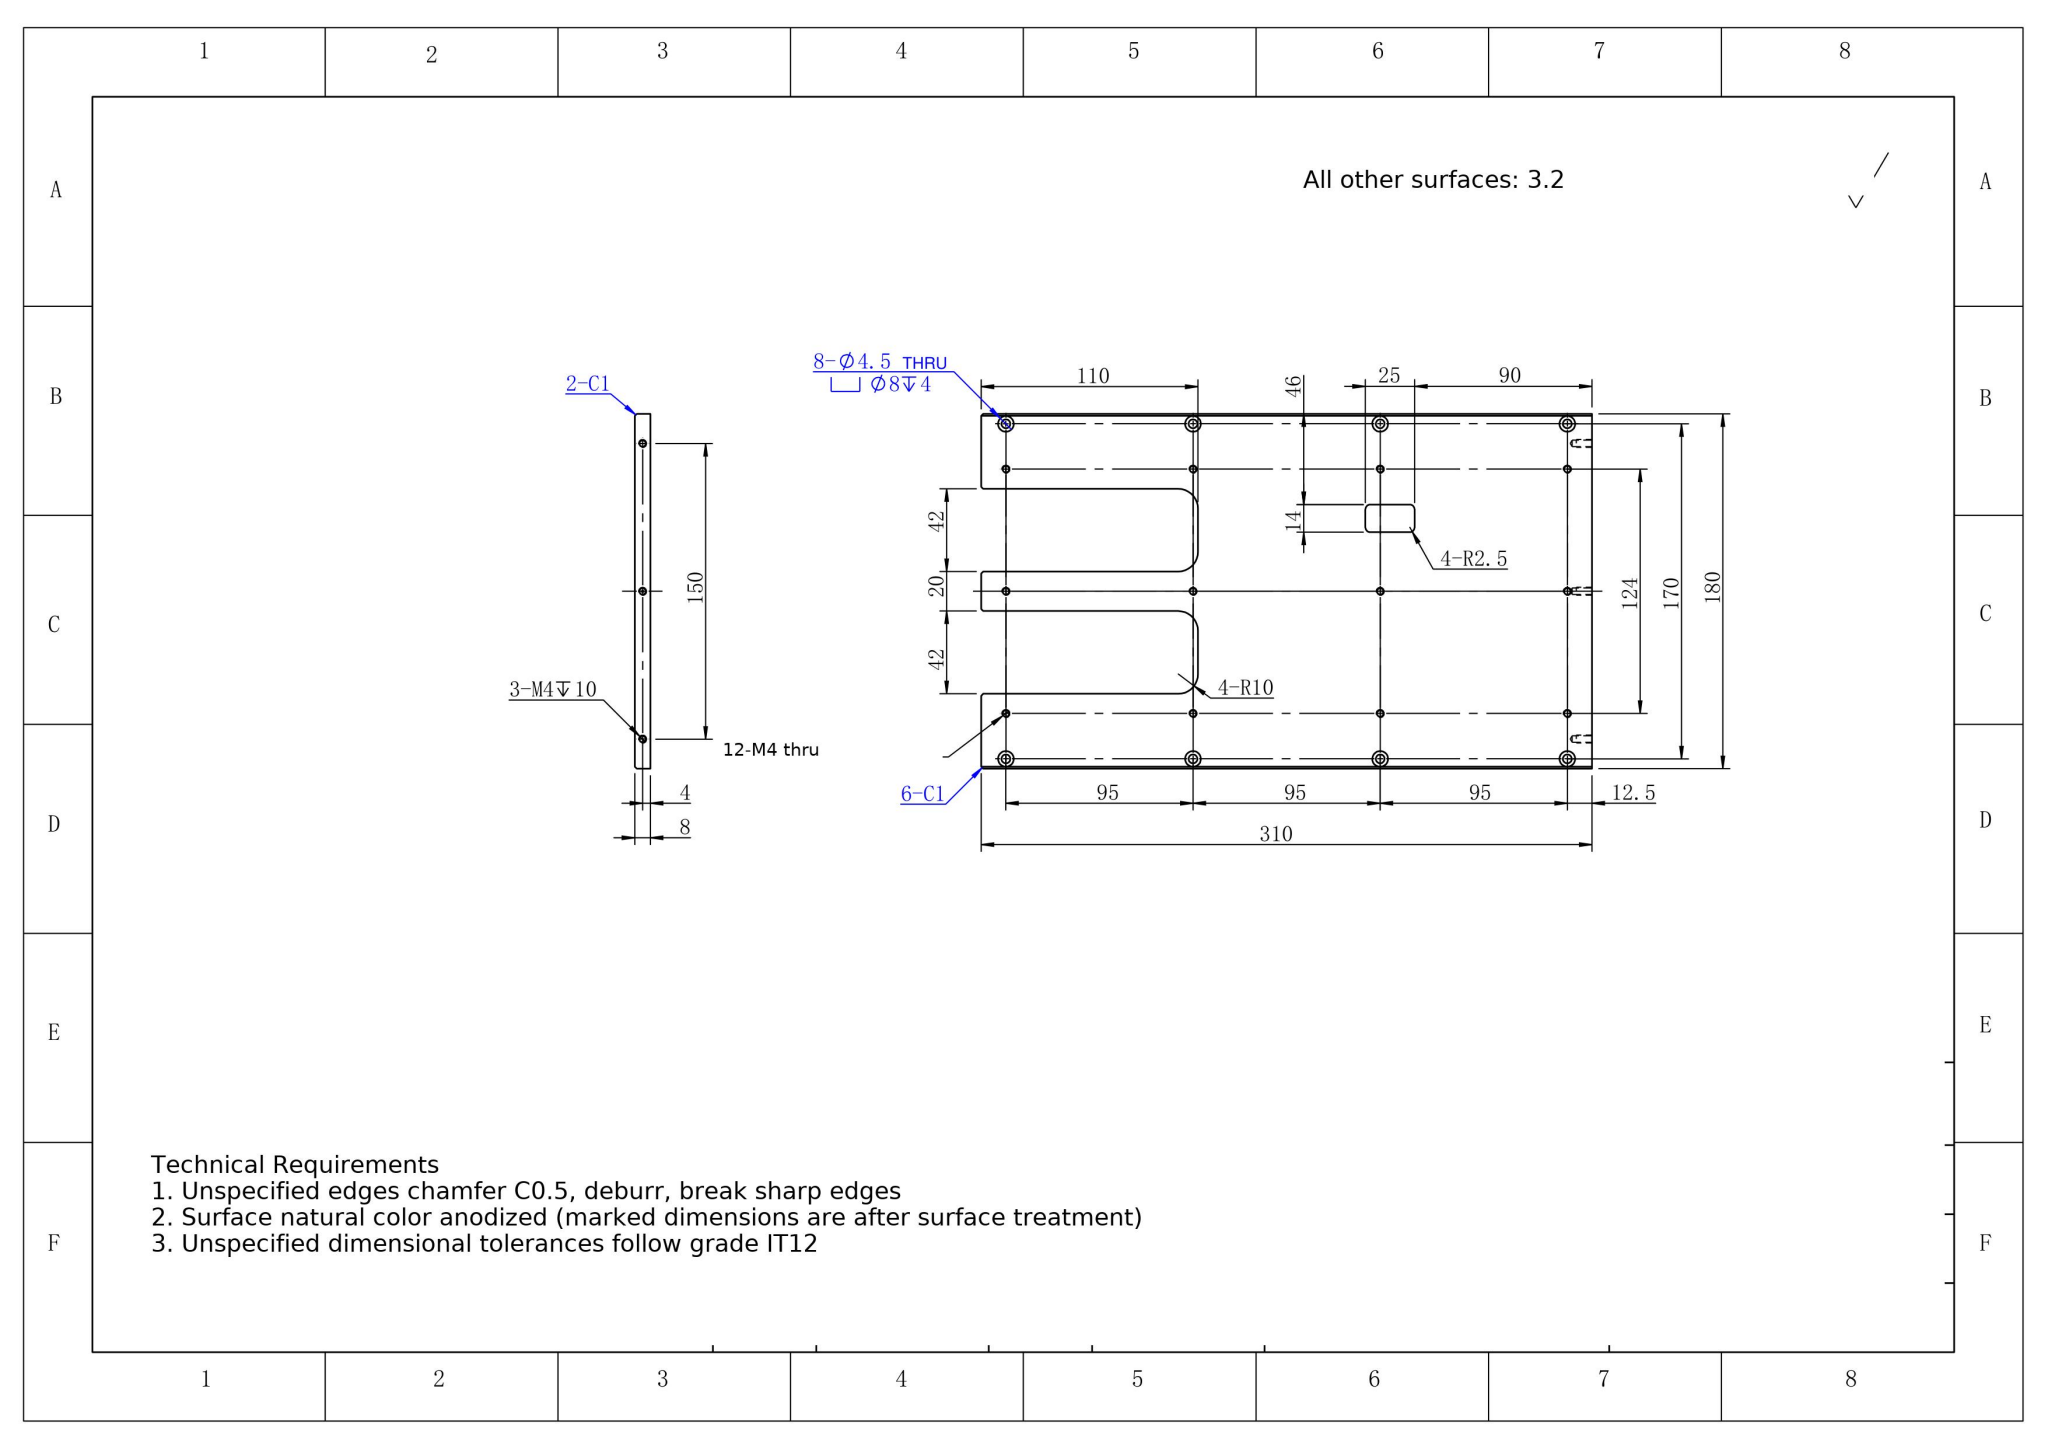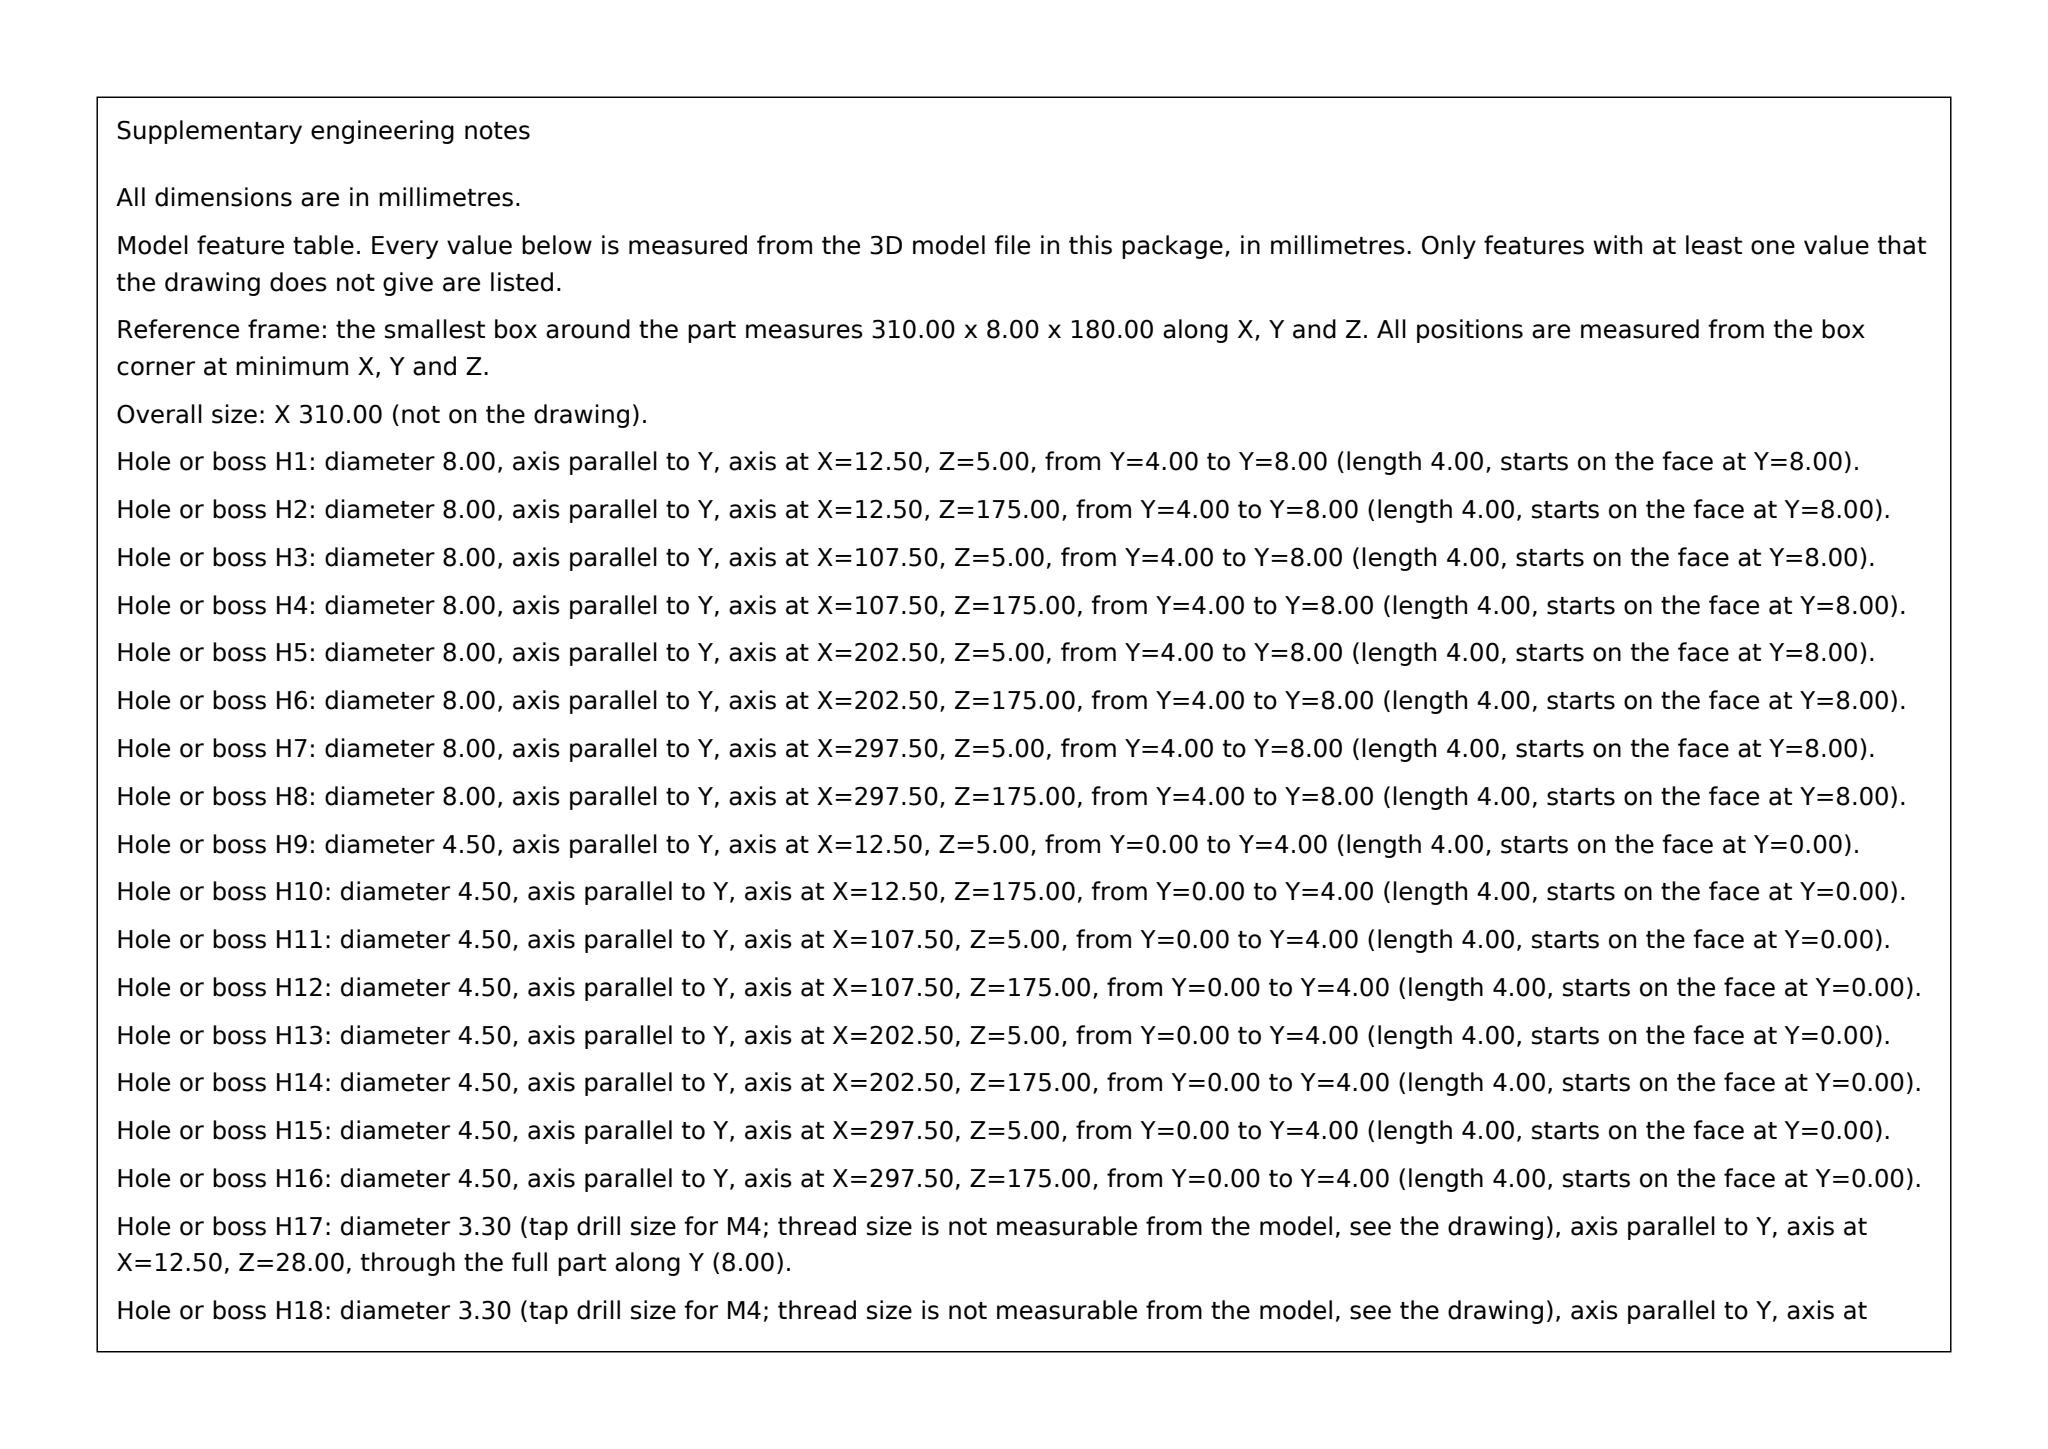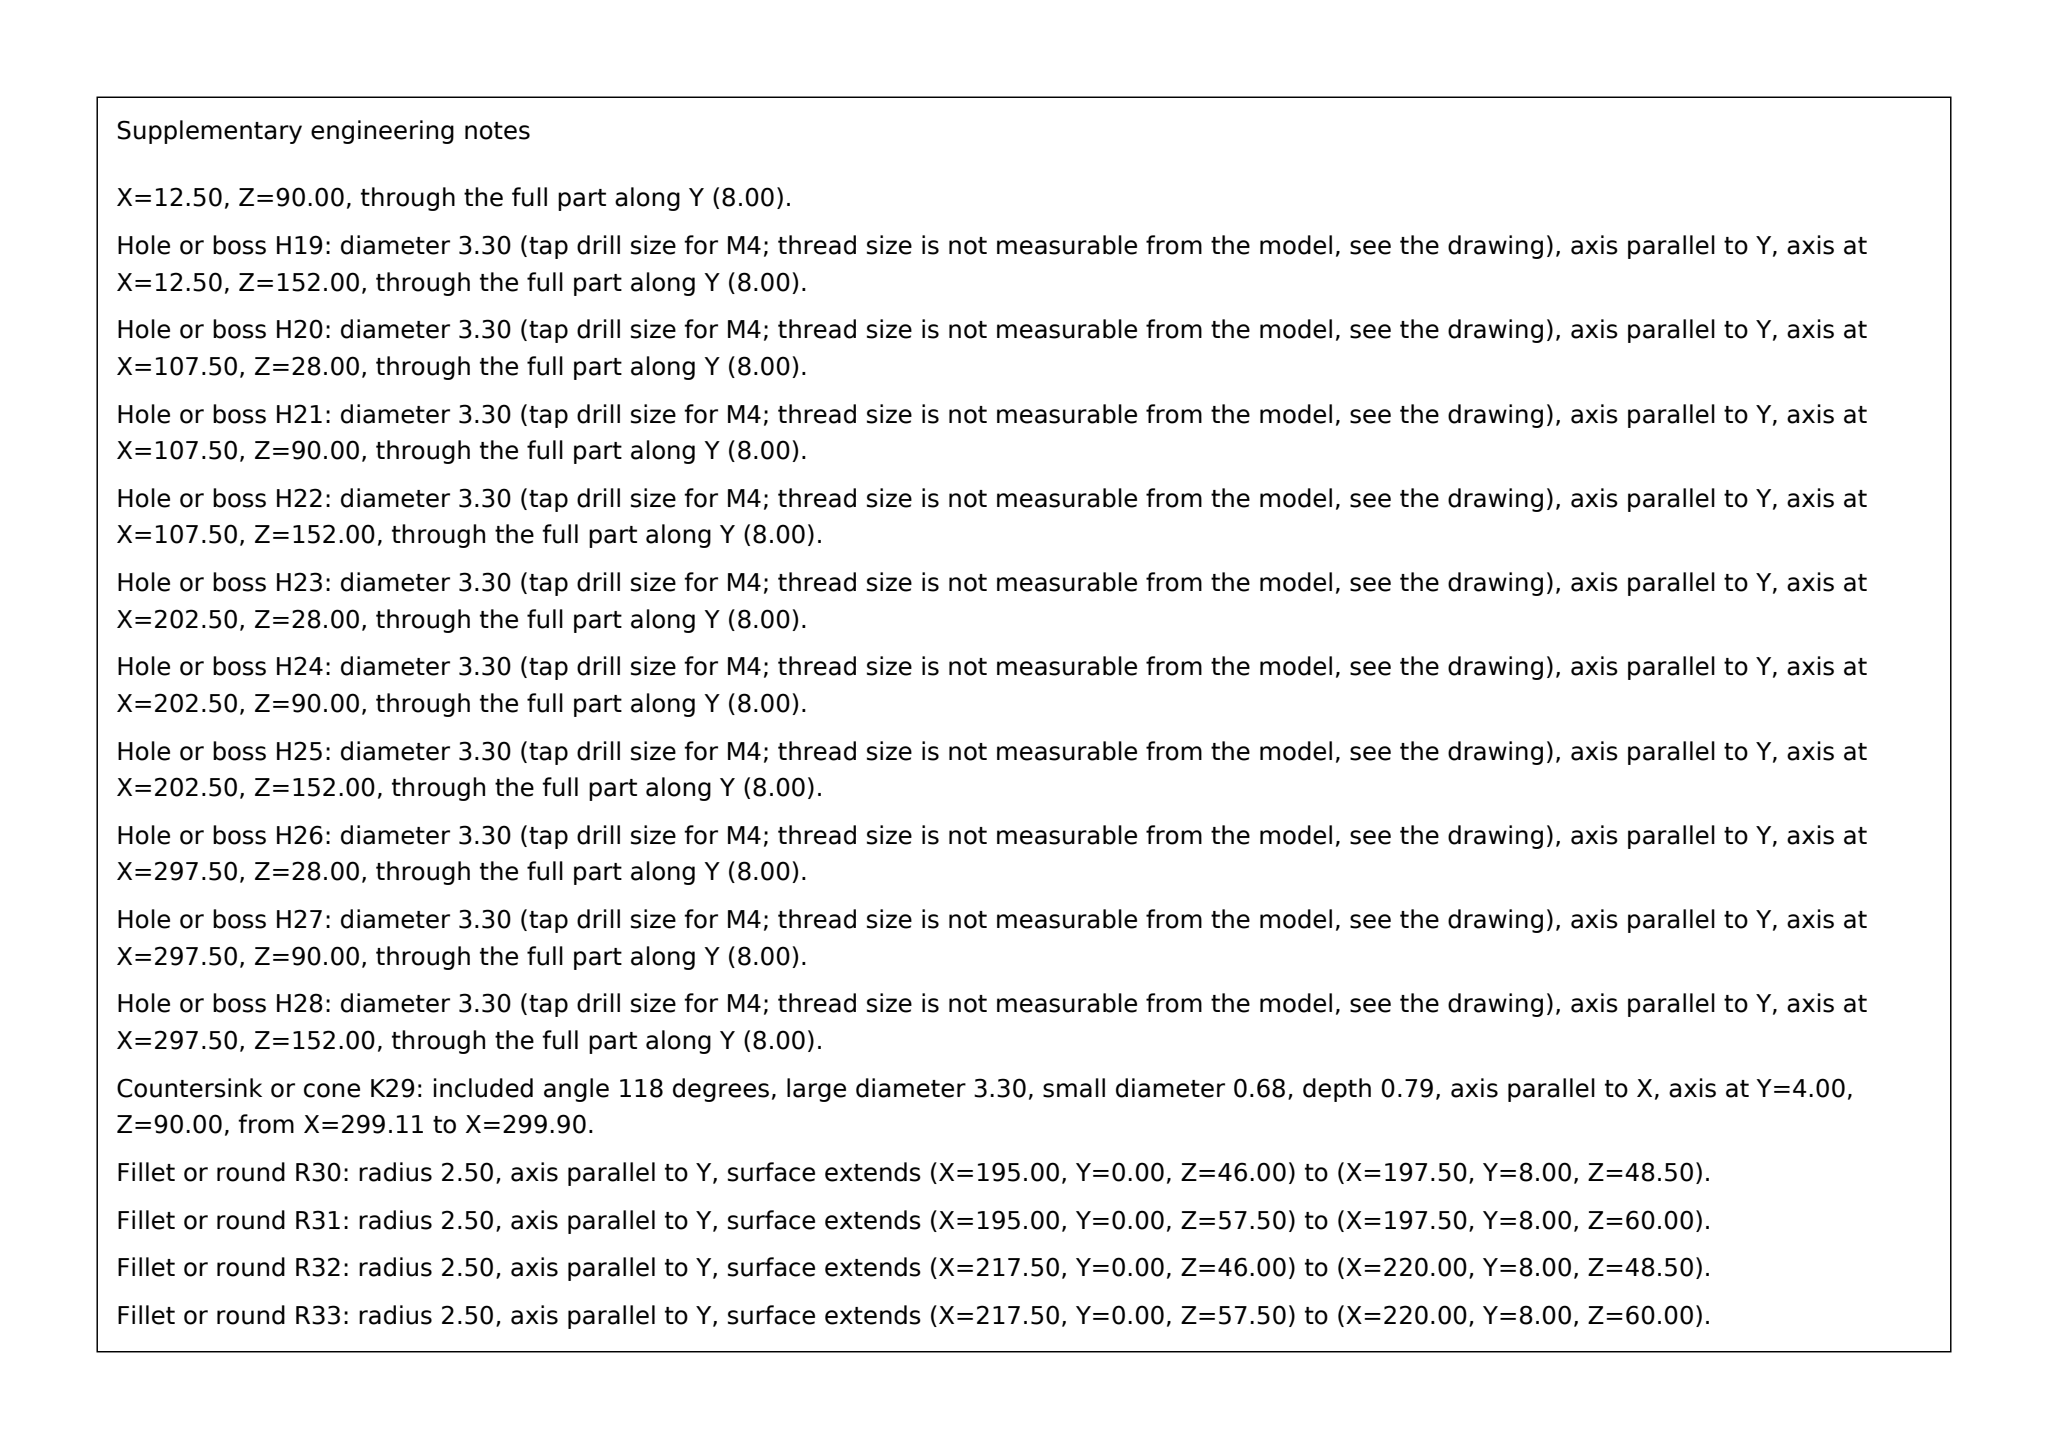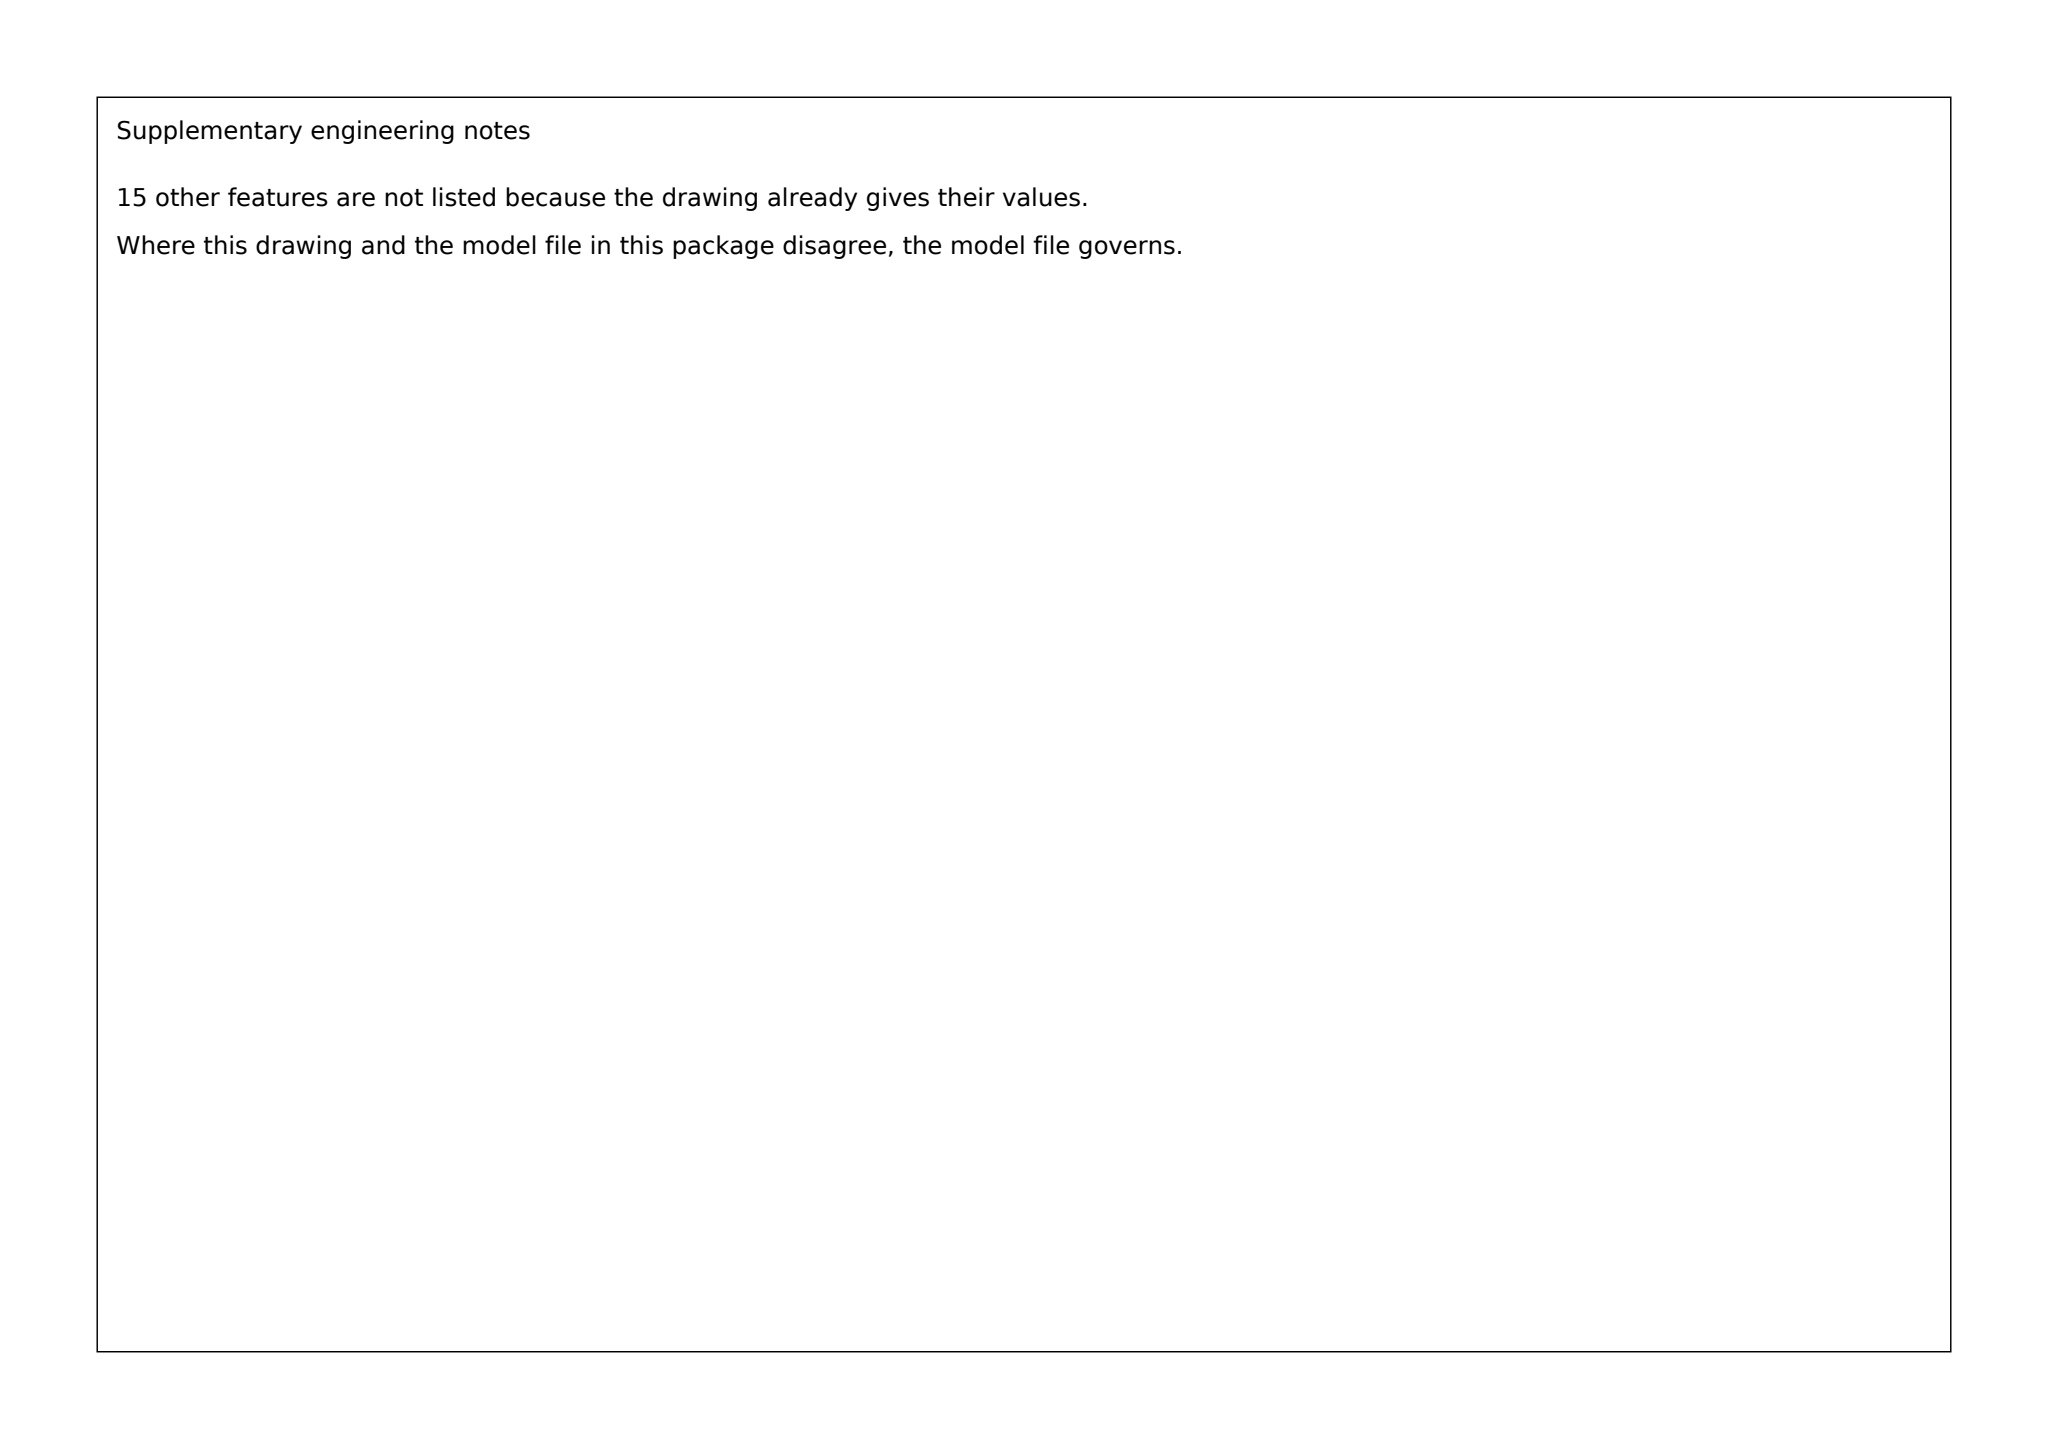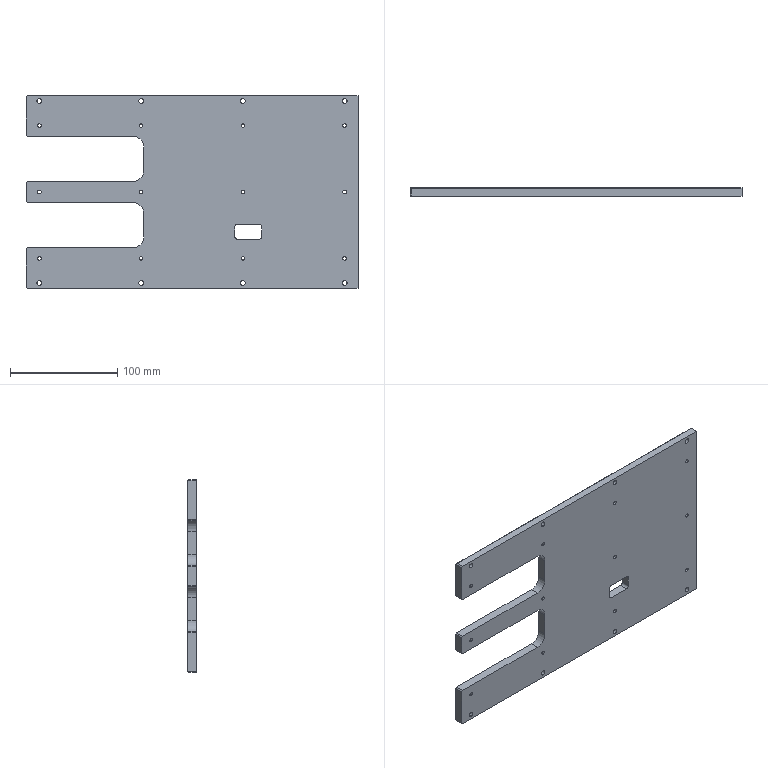Part | SolidWorks | mm | 1 solid | 110 faces | box 310 x 8 x 180 mm | volume 366870 mm3 | cylinder 70 | plane 34 | cone 6 | commonest cylinder face diameters 3.3 x30 8 x16 4.5 x16 20 x4 5 x4